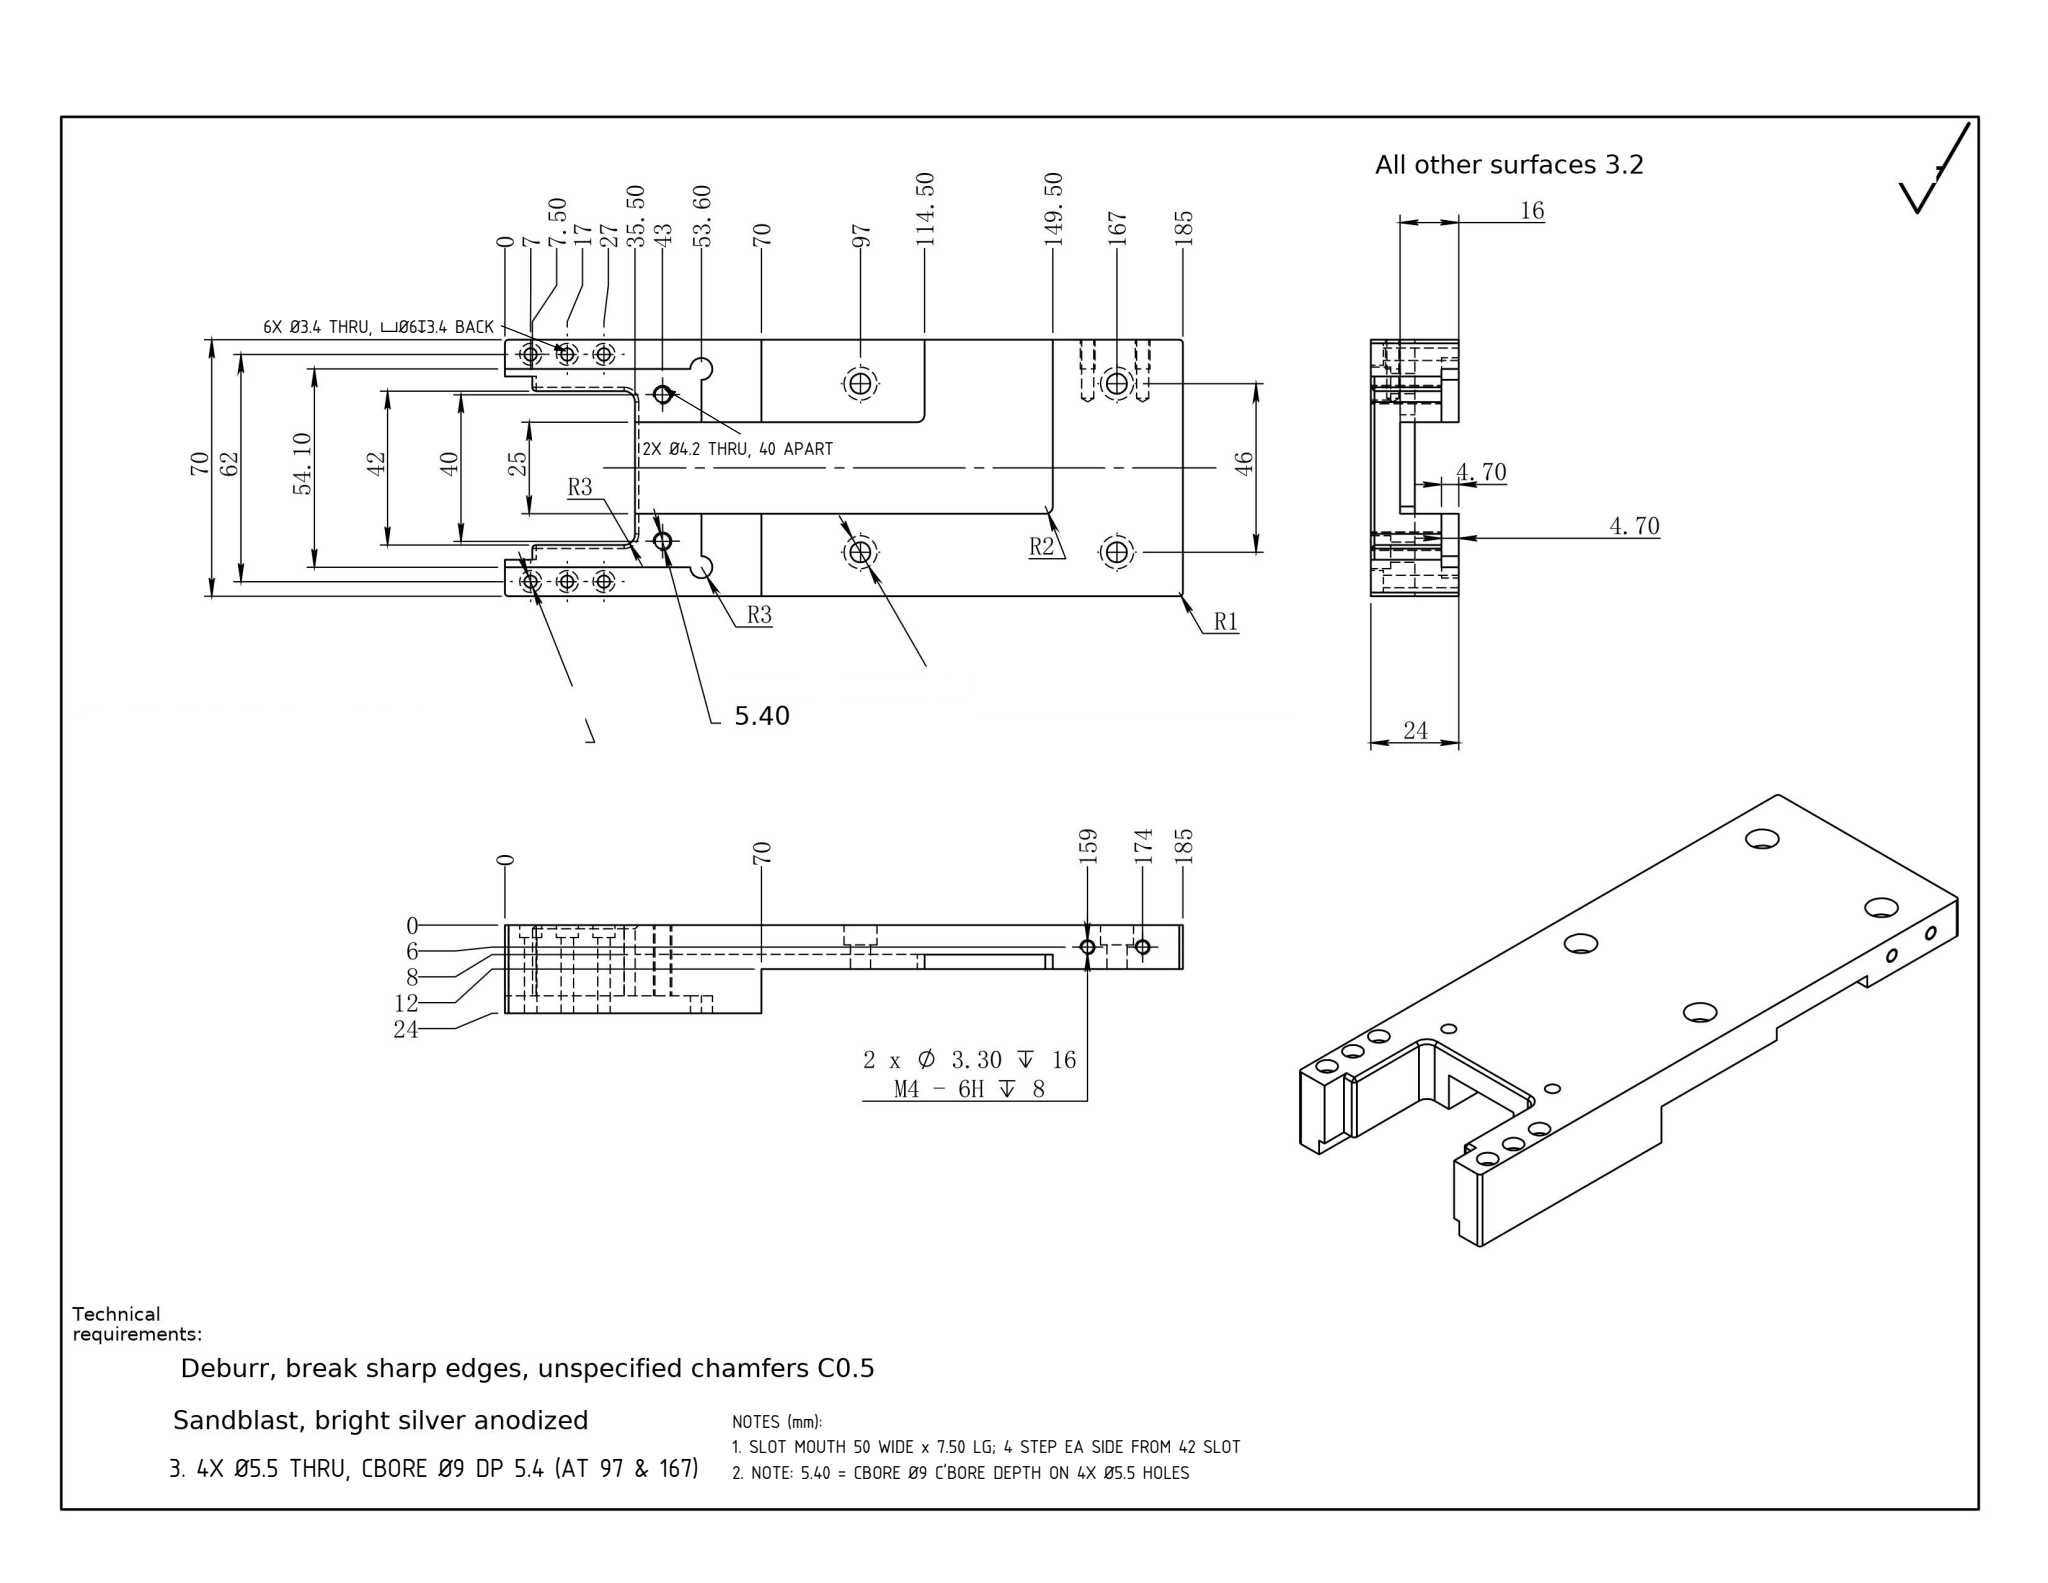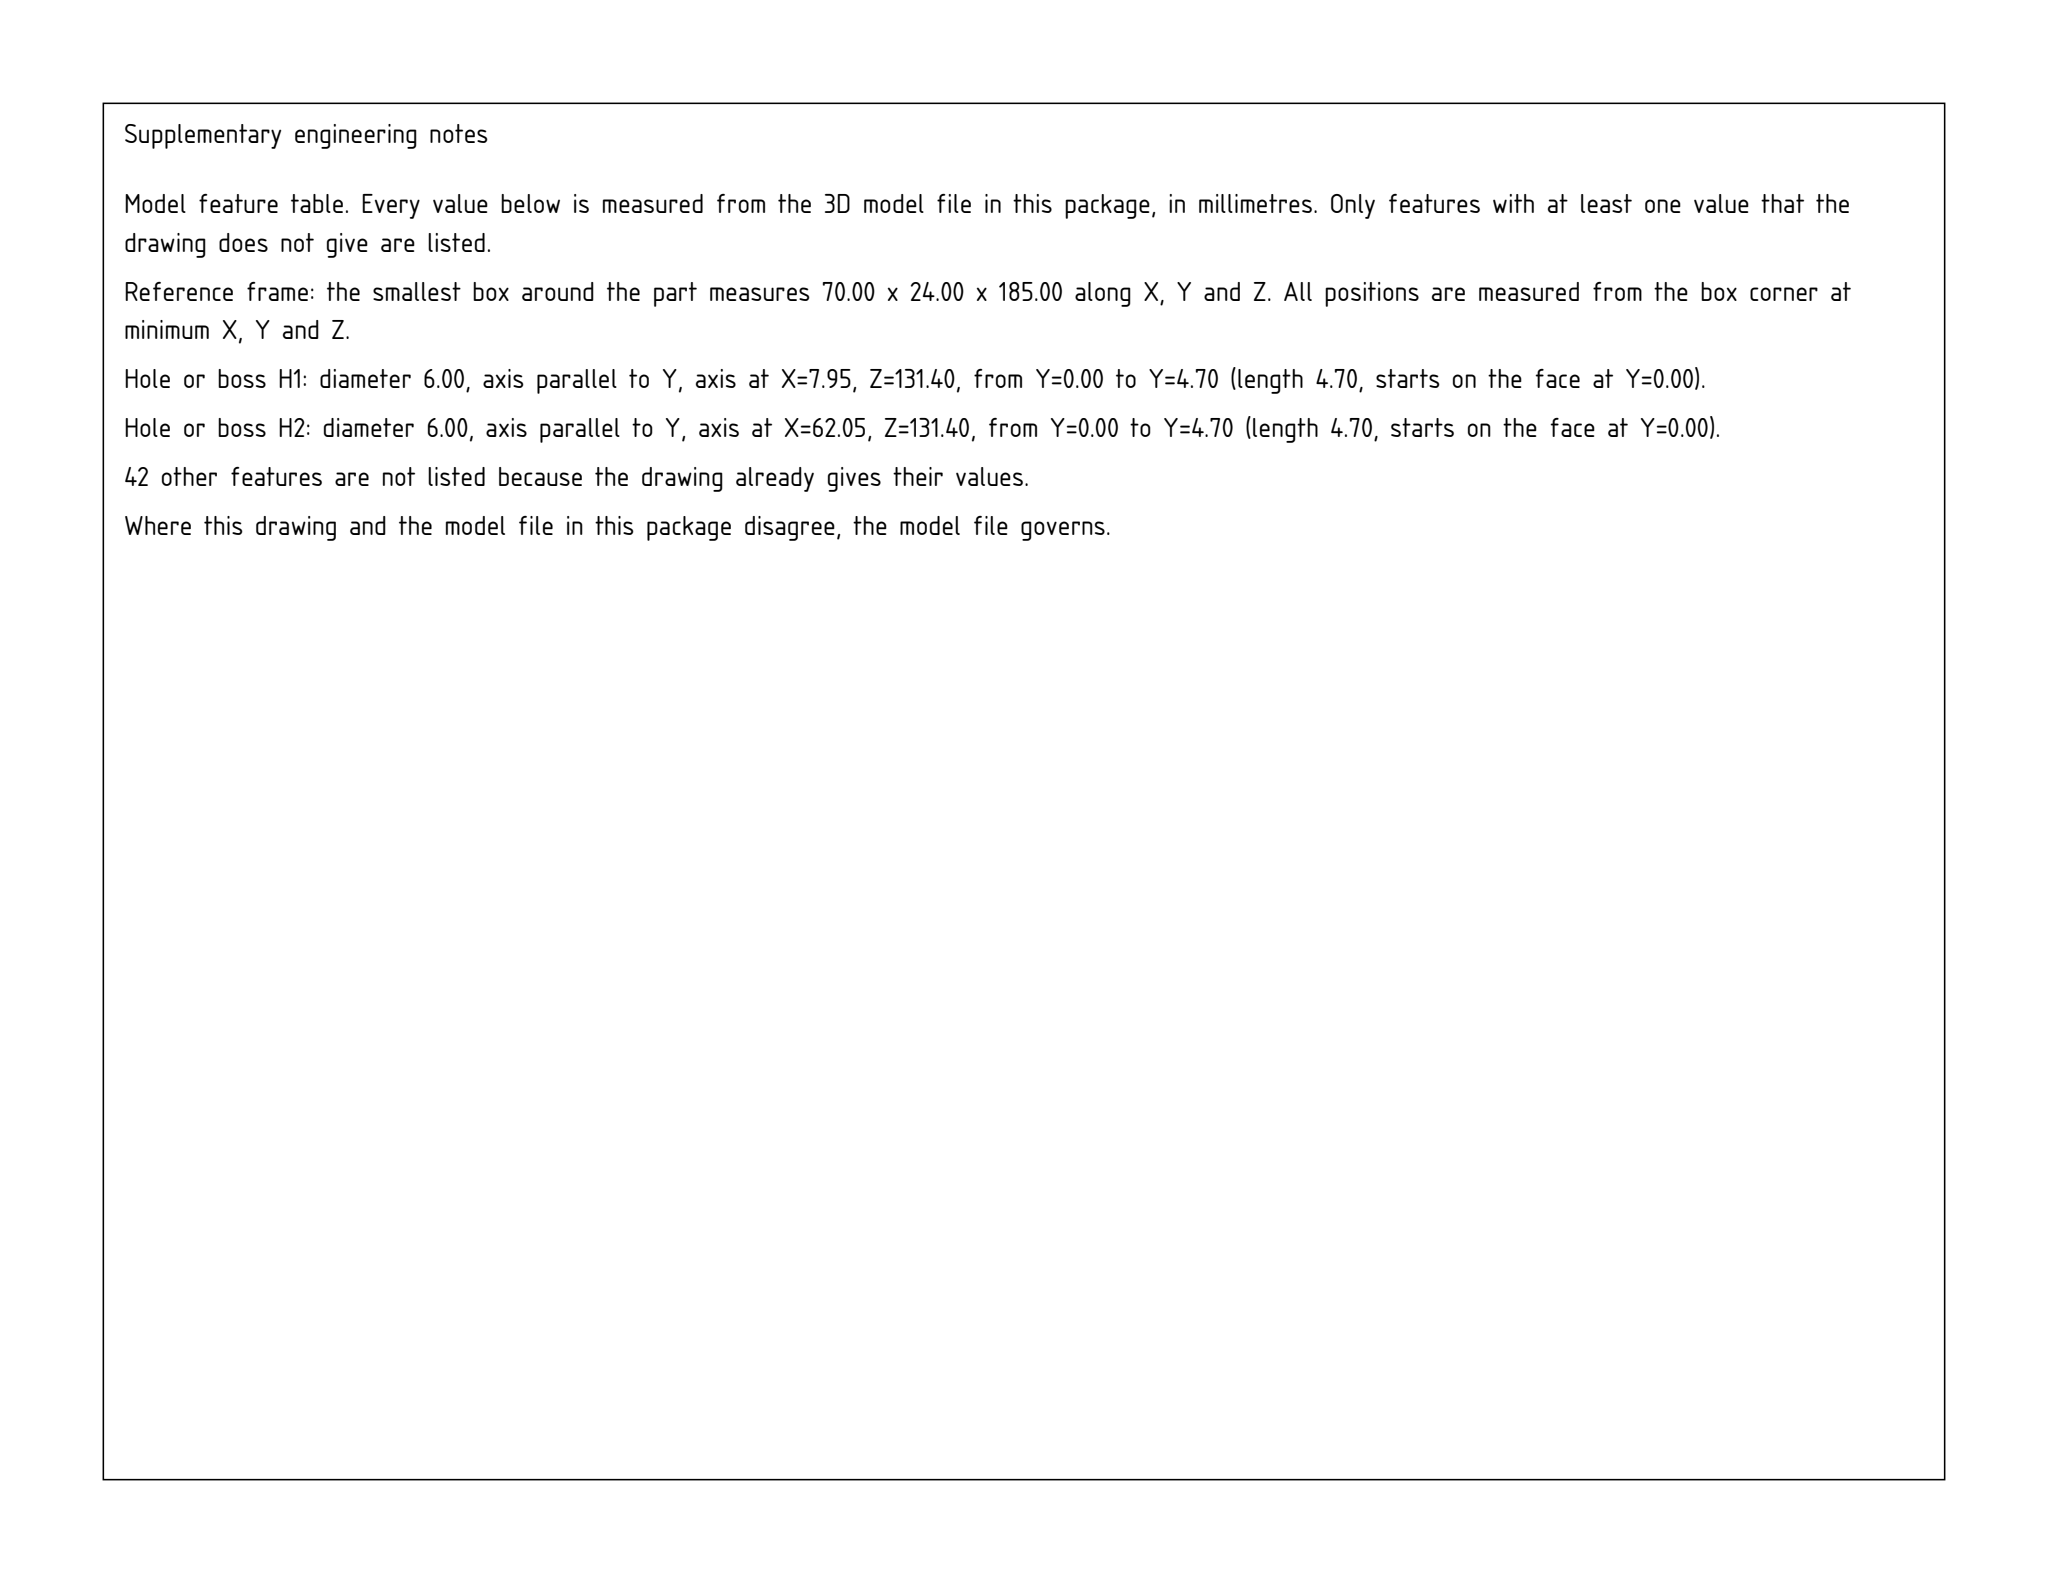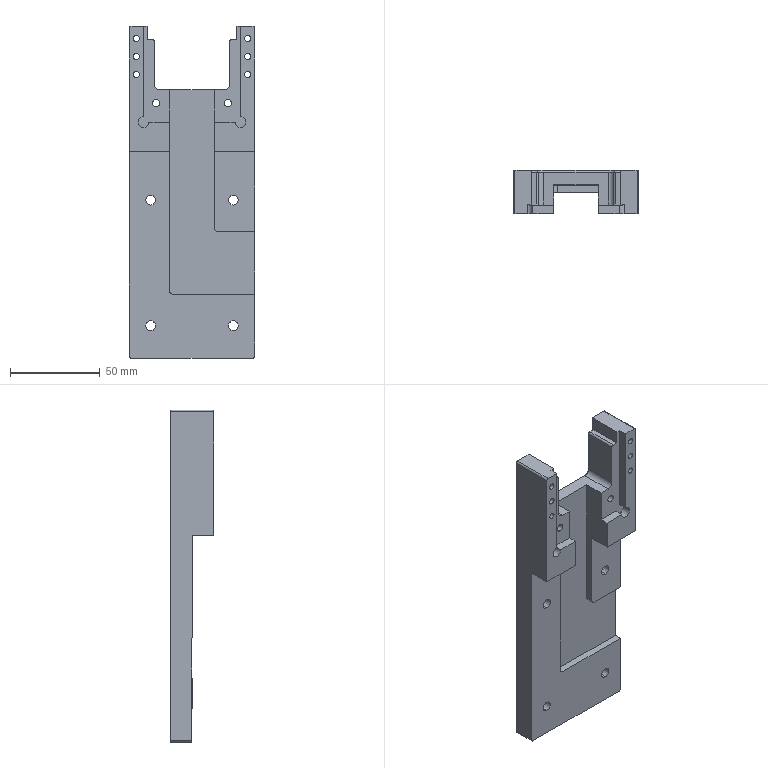Part | SolidWorks | mm | material A6061 | 1 solid | 113 faces | box 70 x 24 x 185 mm | volume 143149 mm3 | cylinder 60 | plane 45 | cone 8 | commonest cylinder face diameters 6 x16 3.4 x12 9 x8 5.5 x8 2 x6 3.3 x4 4.2 x4 4 x2
Drawing notes:
6X Ø3.4 THRU, CBORE Ø6 DP 3.4 FROM BACK FACE | from the solid: Six y-axis bores Ø3.4 y=0-20.6 at x=4/66, z=158/168/178 with Ø6 bore y=20.6-24.0 (back face y=24)
4X Ø5.5 THRU, CBORE Ø9 DP 5.4 (AT 97 & 167) | from the solid: Ø5.5 bores y=12-18.6 at x=12/58, z=18 & 88 (=167 & 97 from datum), Ø9 bores y=18.6-24.0 → 5.4 deep
2X Ø4.2 THRU AT 43; X = 15 & 55, 40 APART | from the solid: Ø4.2 y-axis holes y=4.7-24.0 at x=15 and x=55, z=142 (=43 from datum)
SLOT MOUTH 50 WIDE x 7.50 LG; 4 STEP EA SIDE FROM 42 SLOT | from the solid: Faces x=10 & x=60 (z=176.5-185) vs slot faces x=14 & x=56; step planes z=177.5, x=10-13 and 57-60
NOTE: 5.40 = CBORE Ø9 C'BORE DEPTH ON 4X Ø5.5 HOLES | from the solid: Only 5.4 value in model: Ø9 counterbores y=18.6-24.0 at x=12/58, z=18 & 88
build123d program:
from build123d import *

# Parameters (mm, degrees)
SKETCH1_W                                       = 70
SKETCH1_H                                       = 185
BOSS_EXTRUDE1_DEPTH                             = 12
SKETCH2_W                                       = 54.1
SKETCH2_H                                       = 53.6
CUT_EXTRUDE1_DEPTH                              = 4.7
M5_HEX_SOCKET_HEAD_CAP_SCREW_CBORE1_D           = 5.5
M5_HEX_SOCKET_HEAD_CAP_SCREW_CBORE1_CBORE_D     = 9
M5_HEX_SOCKET_HEAD_CAP_SCREW_CBORE1_CBORE_DEPTH = 5.4
SKETCH9_W                                       = 50
SKETCH9_H                                       = 7.5
CUT_EXTRUDE2_DEPTH                              = 102.771
SKETCH15_W                                      = 42
SKETCH15_H                                      = 28
CUT_EXTRUDE4_DEPTH                              = 102.771
FILLET2_R                                       = 3
SKETCH20_R                                      = 3
CUT_EXTRUDE6_DEPTH                              = 101.766
M5_TAPPED_HOLE1_D                               = 4.2
SKETCH29_W                                      = 115
SKETCH29_H                                      = 12
CUT_EXTRUDE9_DEPTH                              = 117.62
FILLET4_R                                       = 1
FILLET5_R                                       = 1
CUT_EXTRUDE10_DEPTH                             = 100.626
CUT_EXTRUDE10_DEPTH_BACK                        = 4
CHAMFER1_SIZE                                   = 1
M3_HEX_SOCKET_HEAD_CAP_SCREW_CBORE1_D           = 3.4
M3_HEX_SOCKET_HEAD_CAP_SCREW_CBORE1_CBORE_D     = 6
M3_HEX_SOCKET_HEAD_CAP_SCREW_CBORE1_CBORE_DEPTH = 3.4
FILLET6_R                                       = 2
M4_TAPPED_HOLE1_D                               = 3.3
M4_TAPPED_HOLE1_DEPTH                           = 16
M4_TAPPED_HOLE1_TIP                             = 0.9914


with BuildPart() as part:
    # Sketch1 → Boss-Extrude1 (new, symmetric)
    with BuildSketch(Plane(origin=(0, 0, 0), x_dir=(1, 0, 0), z_dir=(0, 1, 0))):
        Rectangle(SKETCH1_W, SKETCH1_H)
    extrude(amount=BOSS_EXTRUDE1_DEPTH, both=True)

    # Sketch2 → Cut-Extrude1 (cut)
    with BuildSketch(Plane(origin=(0, -12, 0), x_dir=(-1, 0, 0), z_dir=(0, -1, 0))):
        with Locations((0, -65.7)):
            Rectangle(SKETCH2_W, SKETCH2_H)
    extrude(amount=-CUT_EXTRUDE1_DEPTH, mode=Mode.SUBTRACT)

    # M5 Hex Socket Head Cap Screw CBORE1 (through all)
    with Locations(Plane(origin=(0, 12, 0), x_dir=(1, 0, 0), z_dir=(0, 1, 0))):
        with Locations((-23, 4.5), (23, 74.5), (23, 4.5), (-23, 74.5)):
            CounterBoreHole(M5_HEX_SOCKET_HEAD_CAP_SCREW_CBORE1_D / 2, M5_HEX_SOCKET_HEAD_CAP_SCREW_CBORE1_CBORE_D / 2, M5_HEX_SOCKET_HEAD_CAP_SCREW_CBORE1_CBORE_DEPTH)

    # Sketch9 → Cut-Extrude2 (cut, through all)
    with BuildSketch(Plane(origin=(0, -12, 0), x_dir=(-1, 0, 0), z_dir=(0, -1, 0))):
        with Locations((0, -88.75)):
            Rectangle(SKETCH9_W, SKETCH9_H)
    extrude(amount=-CUT_EXTRUDE2_DEPTH, mode=Mode.SUBTRACT)

    # Sketch15 → Cut-Extrude4 (cut, through all)
    with BuildSketch(Plane(origin=(0, 12, 0), x_dir=(1, 0, 0), z_dir=(0, 1, 0))):
        with Locations((0, -71)):
            Rectangle(SKETCH15_W, SKETCH15_H)
    extrude(amount=-CUT_EXTRUDE4_DEPTH, mode=Mode.SUBTRACT)

    # Fillet2
    fillet2_edges = [part.edges().sort_by_distance(p)[0] for p in [
        (-21, 2.35, 57),
        (21, 2.35, 57),
    ]]
    fillet(fillet2_edges, radius=FILLET2_R)

    # Sketch20 → Cut-Extrude6 (cut, through all)
    with BuildSketch(Plane(origin=(0, -7.3, 0), x_dir=(-1, 0, 0), z_dir=(0, -1, 0))):
        with Locations((-27.05, -38.9)):
            Circle(SKETCH20_R)
        with Locations((27.05, -38.9)):
            Circle(SKETCH20_R)
    extrude(amount=CUT_EXTRUDE6_DEPTH, mode=Mode.SUBTRACT)

    # M5 Tapped Hole1 (through all)
    with Locations(Plane(origin=(0, -7.3, 0), x_dir=(-1, 0, 0), z_dir=(0, -1, 0))):
        with Locations((-20, -49.5), (20, -49.5)):
            Hole(M5_TAPPED_HOLE1_D / 2)

    # Sketch29 → Cut-Extrude9 (cut, through all)
    with BuildSketch(Plane(origin=(35, 0, 0), x_dir=(0, 0, -1), z_dir=(1, 0, 0))):
        with Locations((35, -6)):
            Rectangle(SKETCH29_W, SKETCH29_H)
    extrude(amount=-CUT_EXTRUDE9_DEPTH, mode=Mode.SUBTRACT)

    # Fillet4
    fillet4_edges = [part.edges().sort_by_distance(p)[0] for p in [
        (35, 0, 92.5),
        (-35, 0, 92.5),
        (21, 2.35, 85),
        (-21, 2.35, 85),
    ]]
    fillet(fillet4_edges, radius=FILLET4_R)

    # Fillet5
    fillet5_edges = [part.edges().sort_by_distance(p)[0] for p in [
        (-35, 6, -92.5),
        (35, 6, -92.5),
    ]]
    fillet(fillet5_edges, radius=FILLET5_R)

    # Sketch30 → Cut-Extrude10 (cut, two sides: drawn at the far end of the back side and taken through both)
    with BuildSketch(Plane.XZ.offset(-CUT_EXTRUDE10_DEPTH_BACK)):
        Polygon((-12.5, -57), (-12.5, 57), (12.5, 57), (12.5, -22), (35, -22), (35, -57), align=None)
    extrude(amount=CUT_EXTRUDE10_DEPTH + CUT_EXTRUDE10_DEPTH_BACK, mode=Mode.SUBTRACT)

    # Chamfer1
    chamfer1_edges = [part.edges().sort_by_distance(p)[0] for p in [
        (-21, 12, 72),
        (20.121, 12, 57.879),
        (-20.121, 12, 57.879),
        (21, 12, 72),
        (23.5, 12, 85),
        (21.293, 12, 84.707),
        (-21.293, 12, 84.707),
        (-23.5, 12, 85),
        (0, 12, 57),
    ]]
    chamfer(chamfer1_edges, length=CHAMFER1_SIZE)

    # M3 Hex Socket Head Cap Screw CBORE1 (through all)
    with Locations(Plane(origin=(0, 12, 0), x_dir=(1, 0, 0), z_dir=(0, 1, 0))):
        with Locations((-31, -65.5), (-31, -75.5), (-31, -85.5)):
            m3_hex_socket_head_cap_screw_cbore1 = CounterBoreHole(M3_HEX_SOCKET_HEAD_CAP_SCREW_CBORE1_D / 2, M3_HEX_SOCKET_HEAD_CAP_SCREW_CBORE1_CBORE_D / 2, M3_HEX_SOCKET_HEAD_CAP_SCREW_CBORE1_CBORE_DEPTH)

    # Mirror1: M3 Hex Socket Head Cap Screw CBORE1 across plane
    add(m3_hex_socket_head_cap_screw_cbore1.mirror(Plane(origin=(0, 0, 0), x_dir=(0, 0, 1), z_dir=(1, 0, 0))), mode=Mode.SUBTRACT)

    # Fillet6
    fillet6_edges = [part.edges().sort_by_distance(p)[0] for p in [
        (-12.5, 2, -57),
        (12.5, 2, -22),
    ]]
    fillet(fillet6_edges, radius=FILLET6_R)

    # M4 Tapped Hole1
    with Locations(Plane(origin=(35, 0, 0), x_dir=(0, 0, -1), z_dir=(1, 0, 0))):
        with Locations((66.5, 6), (81.5, 6)):
            Hole(M4_TAPPED_HOLE1_D / 2, depth=M4_TAPPED_HOLE1_DEPTH)
            with Locations((0, 0, -(M4_TAPPED_HOLE1_DEPTH + M4_TAPPED_HOLE1_TIP / 2))):  # 118° drill point
                Cone(0, M4_TAPPED_HOLE1_D / 2, M4_TAPPED_HOLE1_TIP, mode=Mode.SUBTRACT)


solid = part.part